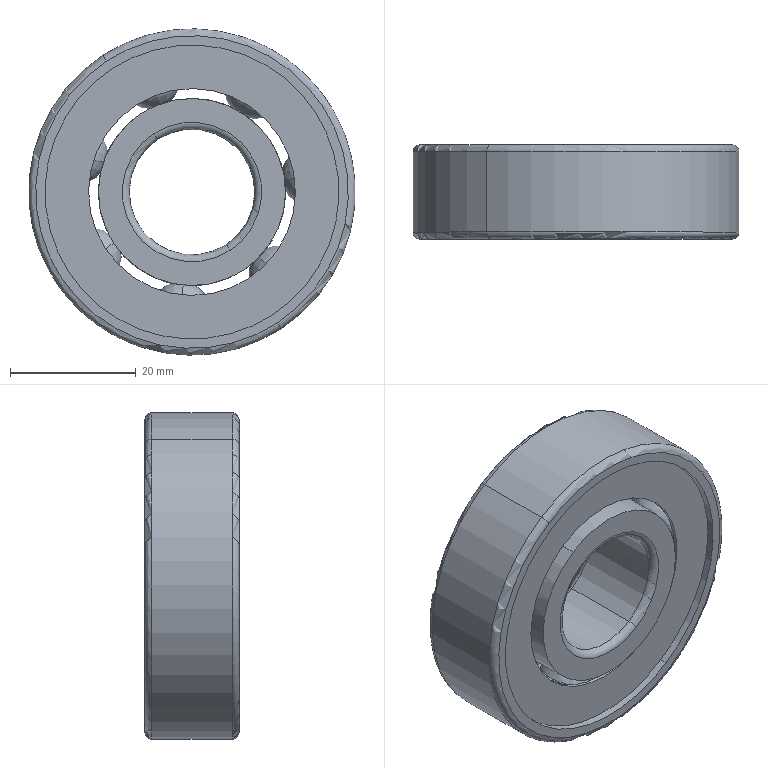Component | SolidWorks | DeepGrooveBallBearing6304-2RZ[GB_T276-94]-1 | 1 solid | 134 faces | volume 15973 mm3 | sphere 56 | torus 32 | cylinder 24 | plane 22 | commonest cylinder face diameters 46.8 x8 32.943 x4 29.8 x4 20 x2 52 x2 40.919 x2 35.681 x2